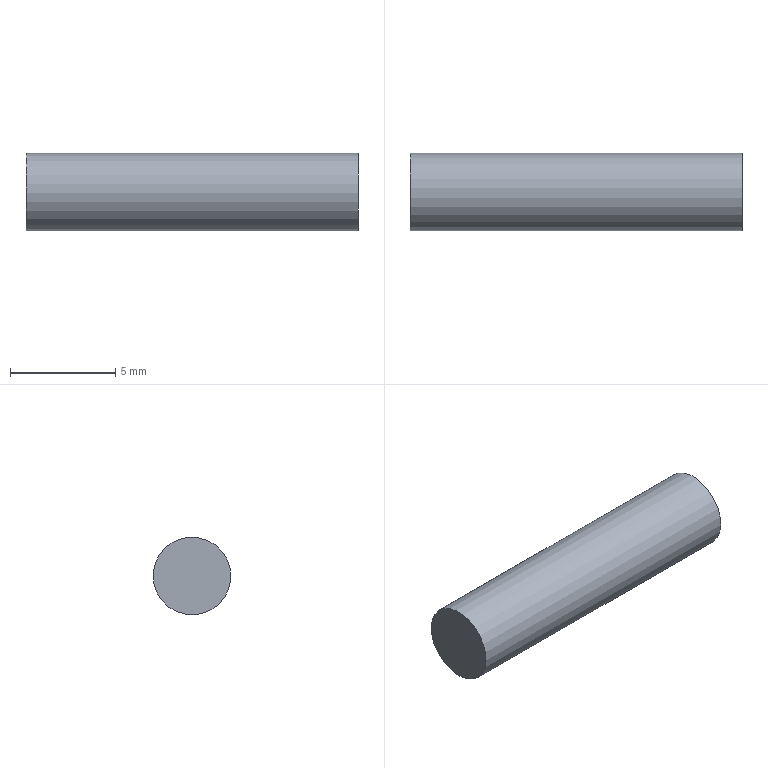Component | NX | SNEIDER_PISTONPIN1 | 1 solid | 3 faces | box 15.75 x 3.68 x 3.68 mm | volume 168 mm3 | plane 2 | cylinder 1 | commonest cylinder face diameters 3.683 x1
STEP:
#1=CARTESIAN_POINT('',(0.,0.,0.));
#2=DIRECTION('',(0.,0.,1.));
#3=DIRECTION('',(1.,0.,0.));
#4=AXIS2_PLACEMENT_3D('',#1,#2,#3);
#5=CARTESIAN_POINT('',(9.271,0.9984,37.971));
#6=VERTEX_POINT('',#5);
#7=CARTESIAN_POINT('',(9.271,0.,36.424));
#8=DIRECTION('',(-1.,0.,0.));
#9=DIRECTION('',(0.,0.5422,0.8403));
#10=AXIS2_PLACEMENT_3D('',#7,#8,#9);
#11=CIRCLE('',#10,1.841);
#12=CARTESIAN_POINT('',(9.271,0.,36.424));
#13=DIRECTION('',(1.,0.,0.));
#14=DIRECTION('',(0.,-0.5422,-0.8403));
#15=AXIS2_PLACEMENT_3D('',#12,#13,#14);
#16=CYLINDRICAL_SURFACE('',#15,1.841);
#17=CARTESIAN_POINT('',(9.425,0.));
#18=DIRECTION('',(-1.,0.));
#19=VECTOR('',#18,1.);
#20=LINE('',#17,#19);
#21=(GEOMETRIC_REPRESENTATION_CONTEXT(2)PARAMETRIC_REPRESENTATION_CONTEXT()REPRESENTATION_CONTEXT('',''));
#22=DEFINITIONAL_REPRESENTATION('',(#20),#21);
#23=PCURVE('',#16,#22);
#24=CARTESIAN_POINT('',(9.271,0.,36.424));
#25=DIRECTION('',(-1.,0.,0.));
#26=DIRECTION('',(0.,0.5422,0.8403));
#27=AXIS2_PLACEMENT_3D('',#24,#25,#26);
#28=PLANE('',#27);
#29=CARTESIAN_POINT('',(0.,0.));
#30=DIRECTION('',(1.,0.));
#31=AXIS2_PLACEMENT_2D('',#29,#30);
#32=CIRCLE('',#31,1.841);
#33=(GEOMETRIC_REPRESENTATION_CONTEXT(2)PARAMETRIC_REPRESENTATION_CONTEXT()REPRESENTATION_CONTEXT('',''));
#34=DEFINITIONAL_REPRESENTATION('',(#32),#33);
#35=PCURVE('',#28,#34);
#36=SURFACE_CURVE('',#11,(#23,#35),.PCURVE_S1.);
#37=EDGE_CURVE('',#6,#6,#36,.T.);
#38=ORIENTED_EDGE('',*,*,#37,.F.);
#39=CARTESIAN_POINT('',(25.019,0.9984,37.971));
#40=VERTEX_POINT('',#39);
#41=CARTESIAN_POINT('',(9.271,0.9984,37.971));
#42=CARTESIAN_POINT('',(25.019,0.9984,37.971));
#43=B_SPLINE_CURVE_WITH_KNOTS('',1,(#41,#42),.UNSPECIFIED.,.F.,.F.,(2,2),(0.,15.748),.PIECEWISE_BEZIER_KNOTS.);
#44=CARTESIAN_POINT('',(9.425,0.));
#45=DIRECTION('',(0.,1.));
#46=VECTOR('',#45,1.);
#47=LINE('',#44,#46);
#48=(GEOMETRIC_REPRESENTATION_CONTEXT(2)PARAMETRIC_REPRESENTATION_CONTEXT()REPRESENTATION_CONTEXT('',''));
#49=DEFINITIONAL_REPRESENTATION('',(#47),#48);
#50=PCURVE('',#16,#49);
#51=CARTESIAN_POINT('',(3.142,0.));
#52=DIRECTION('',(0.,1.));
#53=VECTOR('',#52,1.);
#54=LINE('',#51,#53);
#55=(GEOMETRIC_REPRESENTATION_CONTEXT(2)PARAMETRIC_REPRESENTATION_CONTEXT()REPRESENTATION_CONTEXT('',''));
#56=DEFINITIONAL_REPRESENTATION('',(#54),#55);
#57=PCURVE('',#16,#56);
#58=SEAM_CURVE('',#43,(#50,#57),.PCURVE_S1.);
#59=EDGE_CURVE('',#6,#40,#58,.T.);
#60=ORIENTED_EDGE('',*,*,#59,.T.);
#61=CARTESIAN_POINT('',(25.019,0.,36.424));
#62=DIRECTION('',(-1.,0.,0.));
#63=DIRECTION('',(0.,0.5422,0.8403));
#64=AXIS2_PLACEMENT_3D('',#61,#62,#63);
#65=CIRCLE('',#64,1.841);
#66=CARTESIAN_POINT('',(9.425,15.748));
#67=DIRECTION('',(-1.,0.));
#68=VECTOR('',#67,1.);
#69=LINE('',#66,#68);
#70=(GEOMETRIC_REPRESENTATION_CONTEXT(2)PARAMETRIC_REPRESENTATION_CONTEXT()REPRESENTATION_CONTEXT('',''));
#71=DEFINITIONAL_REPRESENTATION('',(#69),#70);
#72=PCURVE('',#16,#71);
#73=CARTESIAN_POINT('',(25.019,0.,36.424));
#74=DIRECTION('',(-1.,0.,0.));
#75=DIRECTION('',(0.,0.5422,0.8403));
#76=AXIS2_PLACEMENT_3D('',#73,#74,#75);
#77=PLANE('',#76);
#78=CARTESIAN_POINT('',(0.,0.));
#79=DIRECTION('',(1.,0.));
#80=AXIS2_PLACEMENT_2D('',#78,#79);
#81=CIRCLE('',#80,1.841);
#82=(GEOMETRIC_REPRESENTATION_CONTEXT(2)PARAMETRIC_REPRESENTATION_CONTEXT()REPRESENTATION_CONTEXT('',''));
#83=DEFINITIONAL_REPRESENTATION('',(#81),#82);
#84=PCURVE('',#77,#83);
#85=SURFACE_CURVE('',#65,(#72,#84),.PCURVE_S1.);
#86=EDGE_CURVE('',#40,#40,#85,.T.);
#87=ORIENTED_EDGE('',*,*,#86,.T.);
#88=ORIENTED_EDGE('',*,*,#59,.F.);
#89=EDGE_LOOP('',(#38,#60,#87,#88));
#90=FACE_BOUND('',#89,.T.);
#91=ADVANCED_FACE('',(#90),#16,.T.);
#92=ORIENTED_EDGE('',*,*,#37,.T.);
#93=EDGE_LOOP('',(#92));
#94=FACE_BOUND('',#93,.T.);
#95=ADVANCED_FACE('',(#94),#28,.T.);
#96=ORIENTED_EDGE('',*,*,#86,.F.);
#97=EDGE_LOOP('',(#96));
#98=FACE_BOUND('',#97,.T.);
#99=ADVANCED_FACE('',(#98),#77,.F.);
#100=CLOSED_SHELL('',(#91,#95,#99));
#101=MANIFOLD_SOLID_BREP('',#100);
#102=(LENGTH_UNIT()NAMED_UNIT(*)SI_UNIT(.MILLI.,.METRE.));
#103=UNCERTAINTY_MEASURE_WITH_UNIT(LENGTH_MEASURE(0.00001),#102,'','');
#104=(NAMED_UNIT(*)PLANE_ANGLE_UNIT()SI_UNIT($,.RADIAN.));
#105=(NAMED_UNIT(*)SI_UNIT($,.STERADIAN.)SOLID_ANGLE_UNIT());
#106=(GEOMETRIC_REPRESENTATION_CONTEXT(3)GLOBAL_UNCERTAINTY_ASSIGNED_CONTEXT((#103))GLOBAL_UNIT_ASSIGNED_CONTEXT((#102,#104,#105))REPRESENTATION_CONTEXT('',''));
#107=ADVANCED_BREP_SHAPE_REPRESENTATION('',(#4,#101),#106);